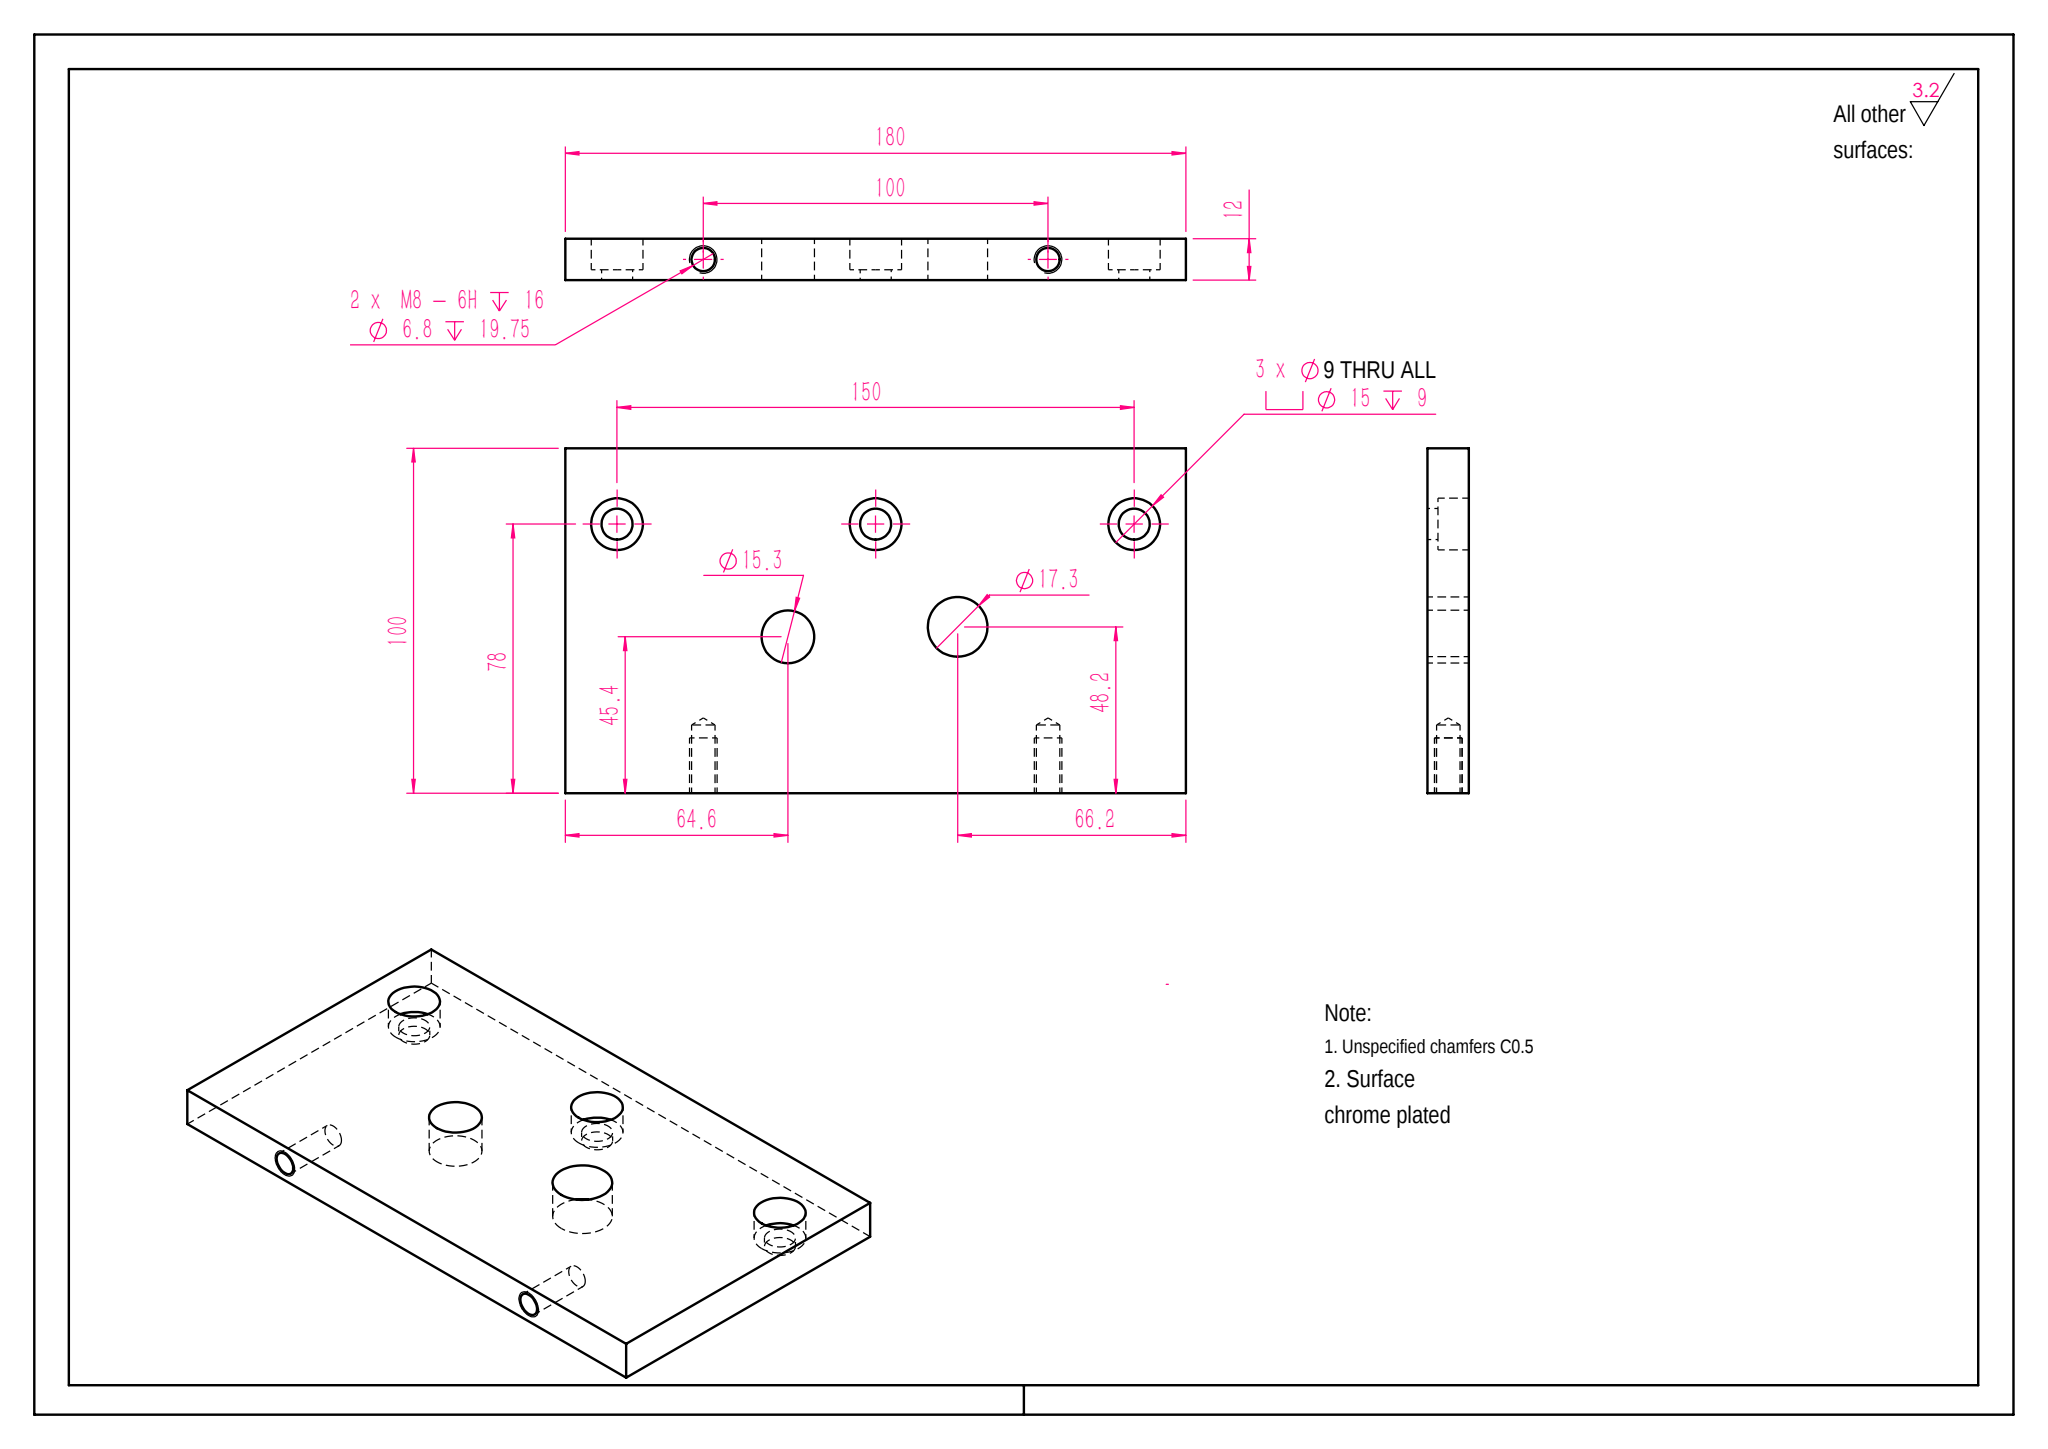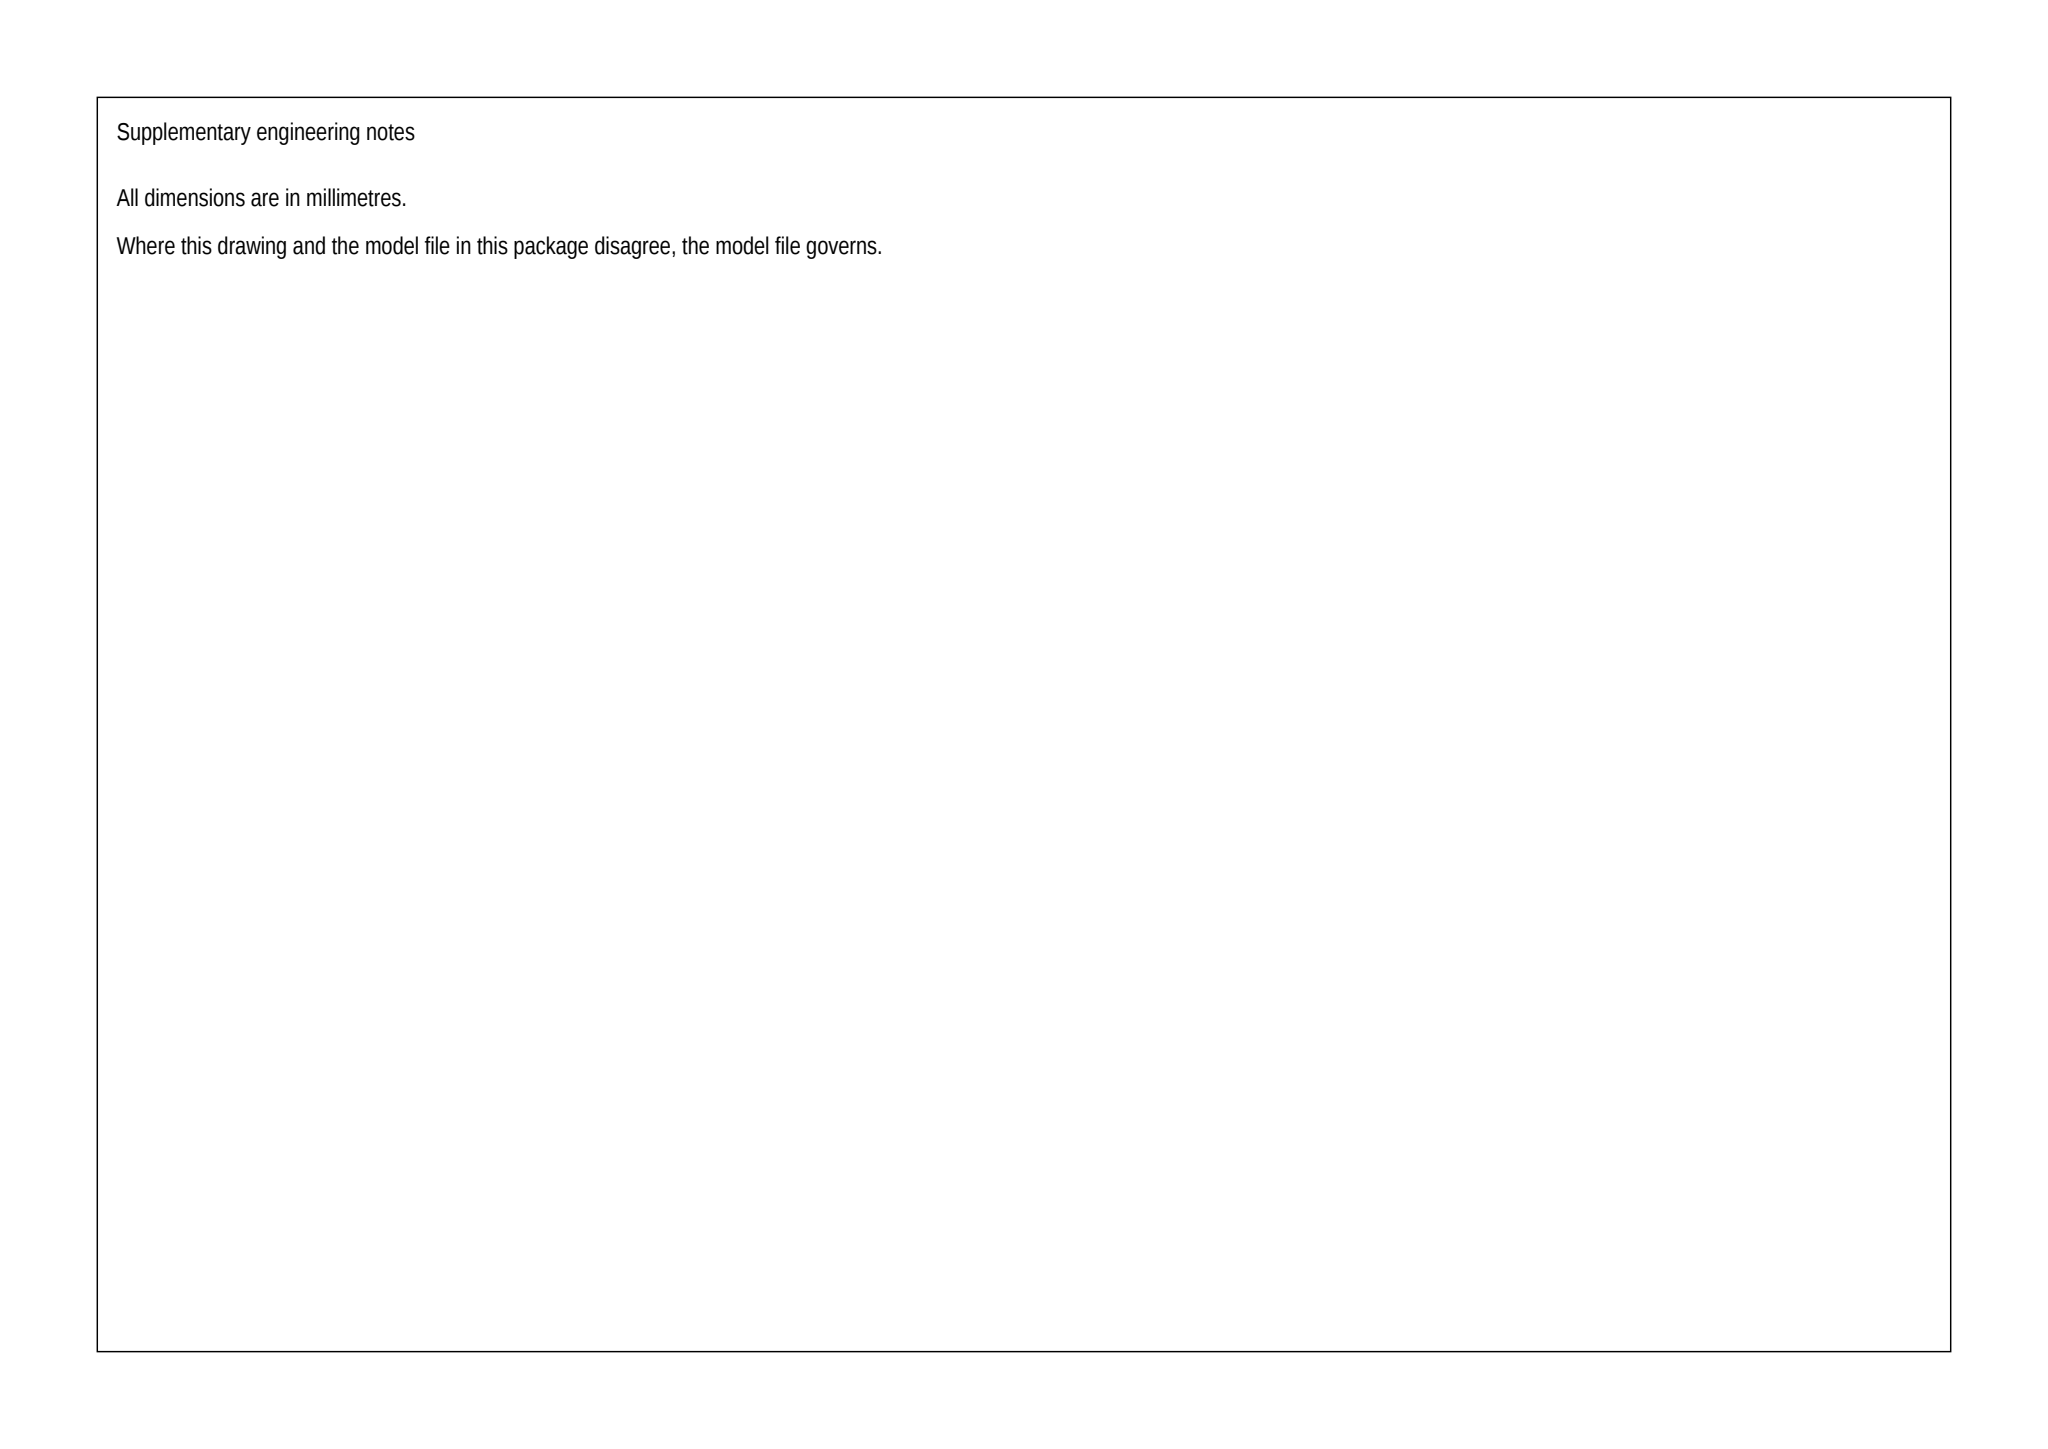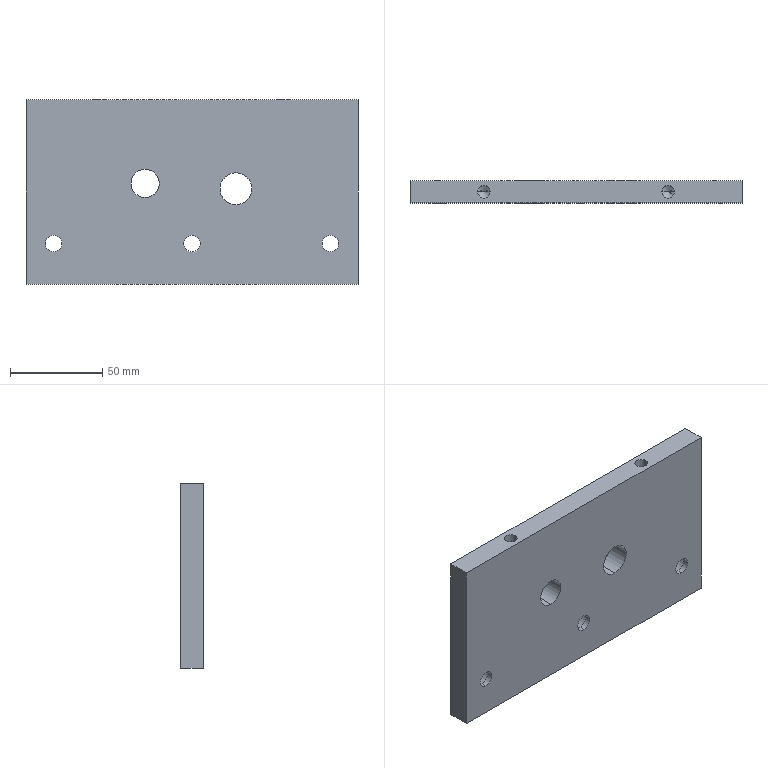Part | SolidWorks | mm | 1 solid | 33 faces | box 180 x 12 x 100 mm | volume 204140 mm3 | cylinder 20 | plane 9 | cone 4 | commonest cylinder face diameters 15 x6 9 x6 6.8 x4 15.312 x2 17.305 x2
build123d program:
from build123d import *

# Parameters (mm, degrees)
SKETCH1_W                                            = 180
SKETCH1_H                                            = 12
BOSS_EXTRUDE1_DEPTH                                  = 100
M8_TAPPED_HOLE1_D                                    = 6.8
M8_TAPPED_HOLE1_DEPTH                                = 19.75
M8_TAPPED_HOLE1_TIP                                  = 2.043
HOLE_SIZE_ACCORDING_TO_HEX_SOCKET_HEAD_C_D           = 9
HOLE_SIZE_ACCORDING_TO_HEX_SOCKET_HEAD_C_CBORE_D     = 15
HOLE_SIZE_ACCORDING_TO_HEX_SOCKET_HEAD_C_CBORE_DEPTH = 9
SKETCH8_R                                            = 7.656
SKETCH8_R_2                                          = 8.653
CUT_EXTRUDE1_DEPTH                                   = 80


with BuildPart() as part:
    # Sketch1 → Boss-Extrude1 (new body)
    with BuildSketch(Plane.XY):
        Rectangle(SKETCH1_W, SKETCH1_H)
    extrude(amount=BOSS_EXTRUDE1_DEPTH)

    # M8 Tapped Hole1
    with Locations(Plane.XY.offset(100)):
        with Locations((-50, 0), (50, 0)):
            Hole(M8_TAPPED_HOLE1_D / 2, depth=M8_TAPPED_HOLE1_DEPTH)
            with Locations((0, 0, -(M8_TAPPED_HOLE1_DEPTH + M8_TAPPED_HOLE1_TIP / 2))):  # 118° drill point
                Cone(0, M8_TAPPED_HOLE1_D / 2, M8_TAPPED_HOLE1_TIP, mode=Mode.SUBTRACT)

    # Hole Size according to Hex Socket Head C (through all)
    with Locations(Plane(origin=(0, 6, 0), x_dir=(1, 0, 0), z_dir=(0, 1, 0))):
        with Locations((-75, -22), (0, -22), (75, -22)):
            CounterBoreHole(HOLE_SIZE_ACCORDING_TO_HEX_SOCKET_HEAD_C_D / 2, HOLE_SIZE_ACCORDING_TO_HEX_SOCKET_HEAD_C_CBORE_D / 2, HOLE_SIZE_ACCORDING_TO_HEX_SOCKET_HEAD_C_CBORE_DEPTH)

    # Sketch8 → Cut-Extrude1 (cut)
    with BuildSketch(Plane(origin=(0, 6, 0), x_dir=(1, 0, 0), z_dir=(0, 1, 0))):
        with Locations(Location((-25.422, -54.638, 0), (0, 0, 270))):
            Circle(SKETCH8_R)
        with Locations(Location((23.795, -51.79, 0), (0, 0, 270))):
            Circle(SKETCH8_R_2)
    extrude(amount=-CUT_EXTRUDE1_DEPTH, mode=Mode.SUBTRACT)


solid = part.part